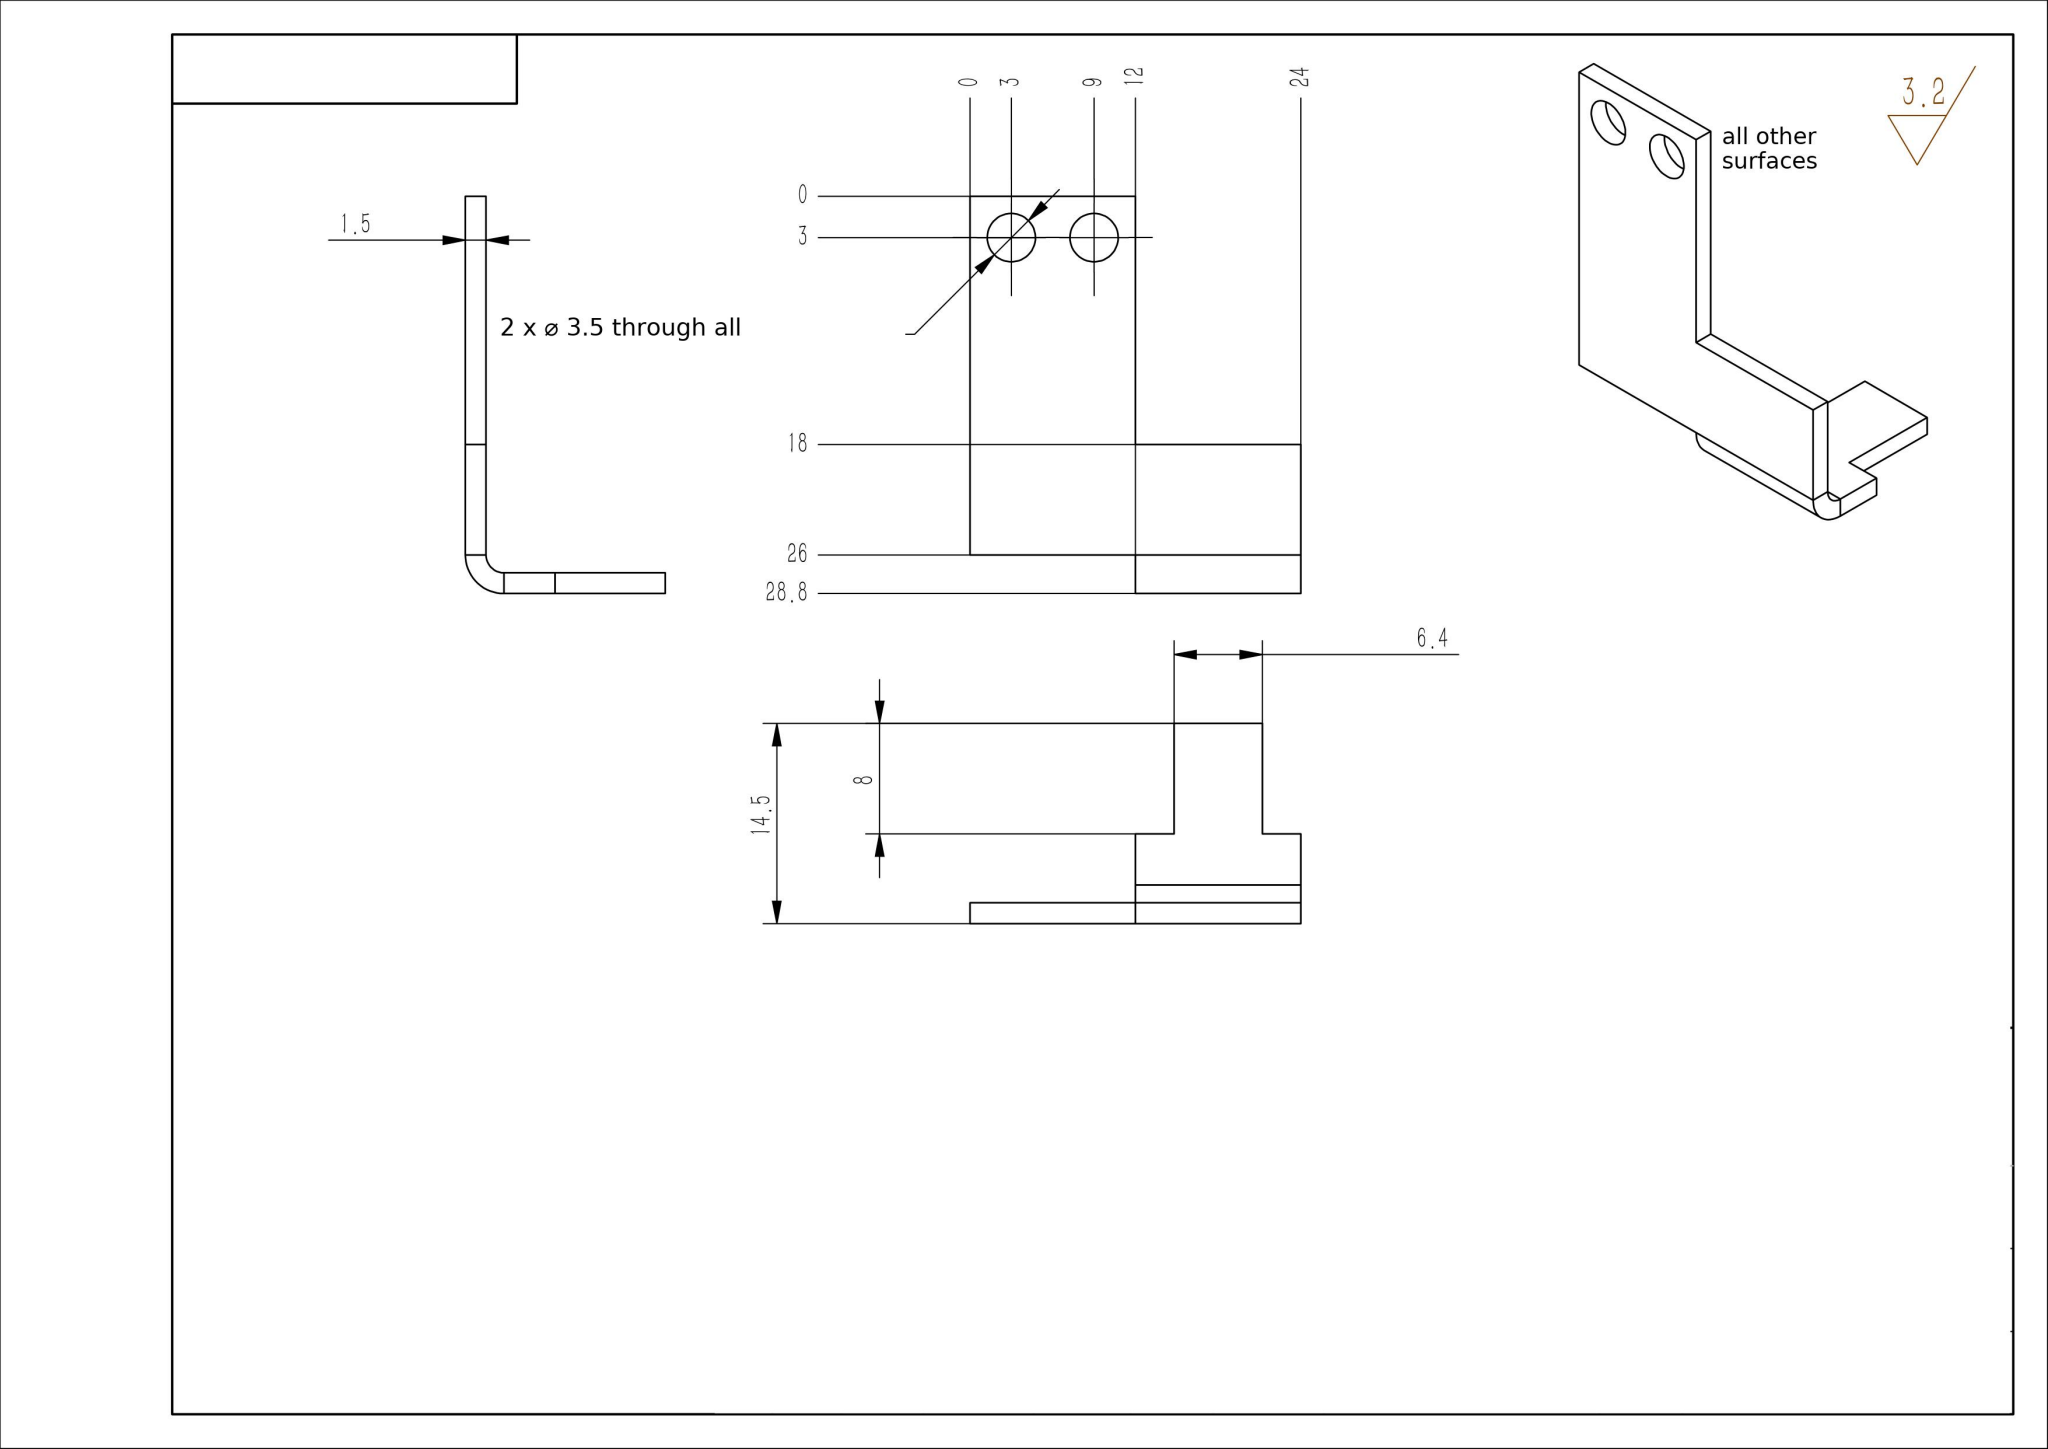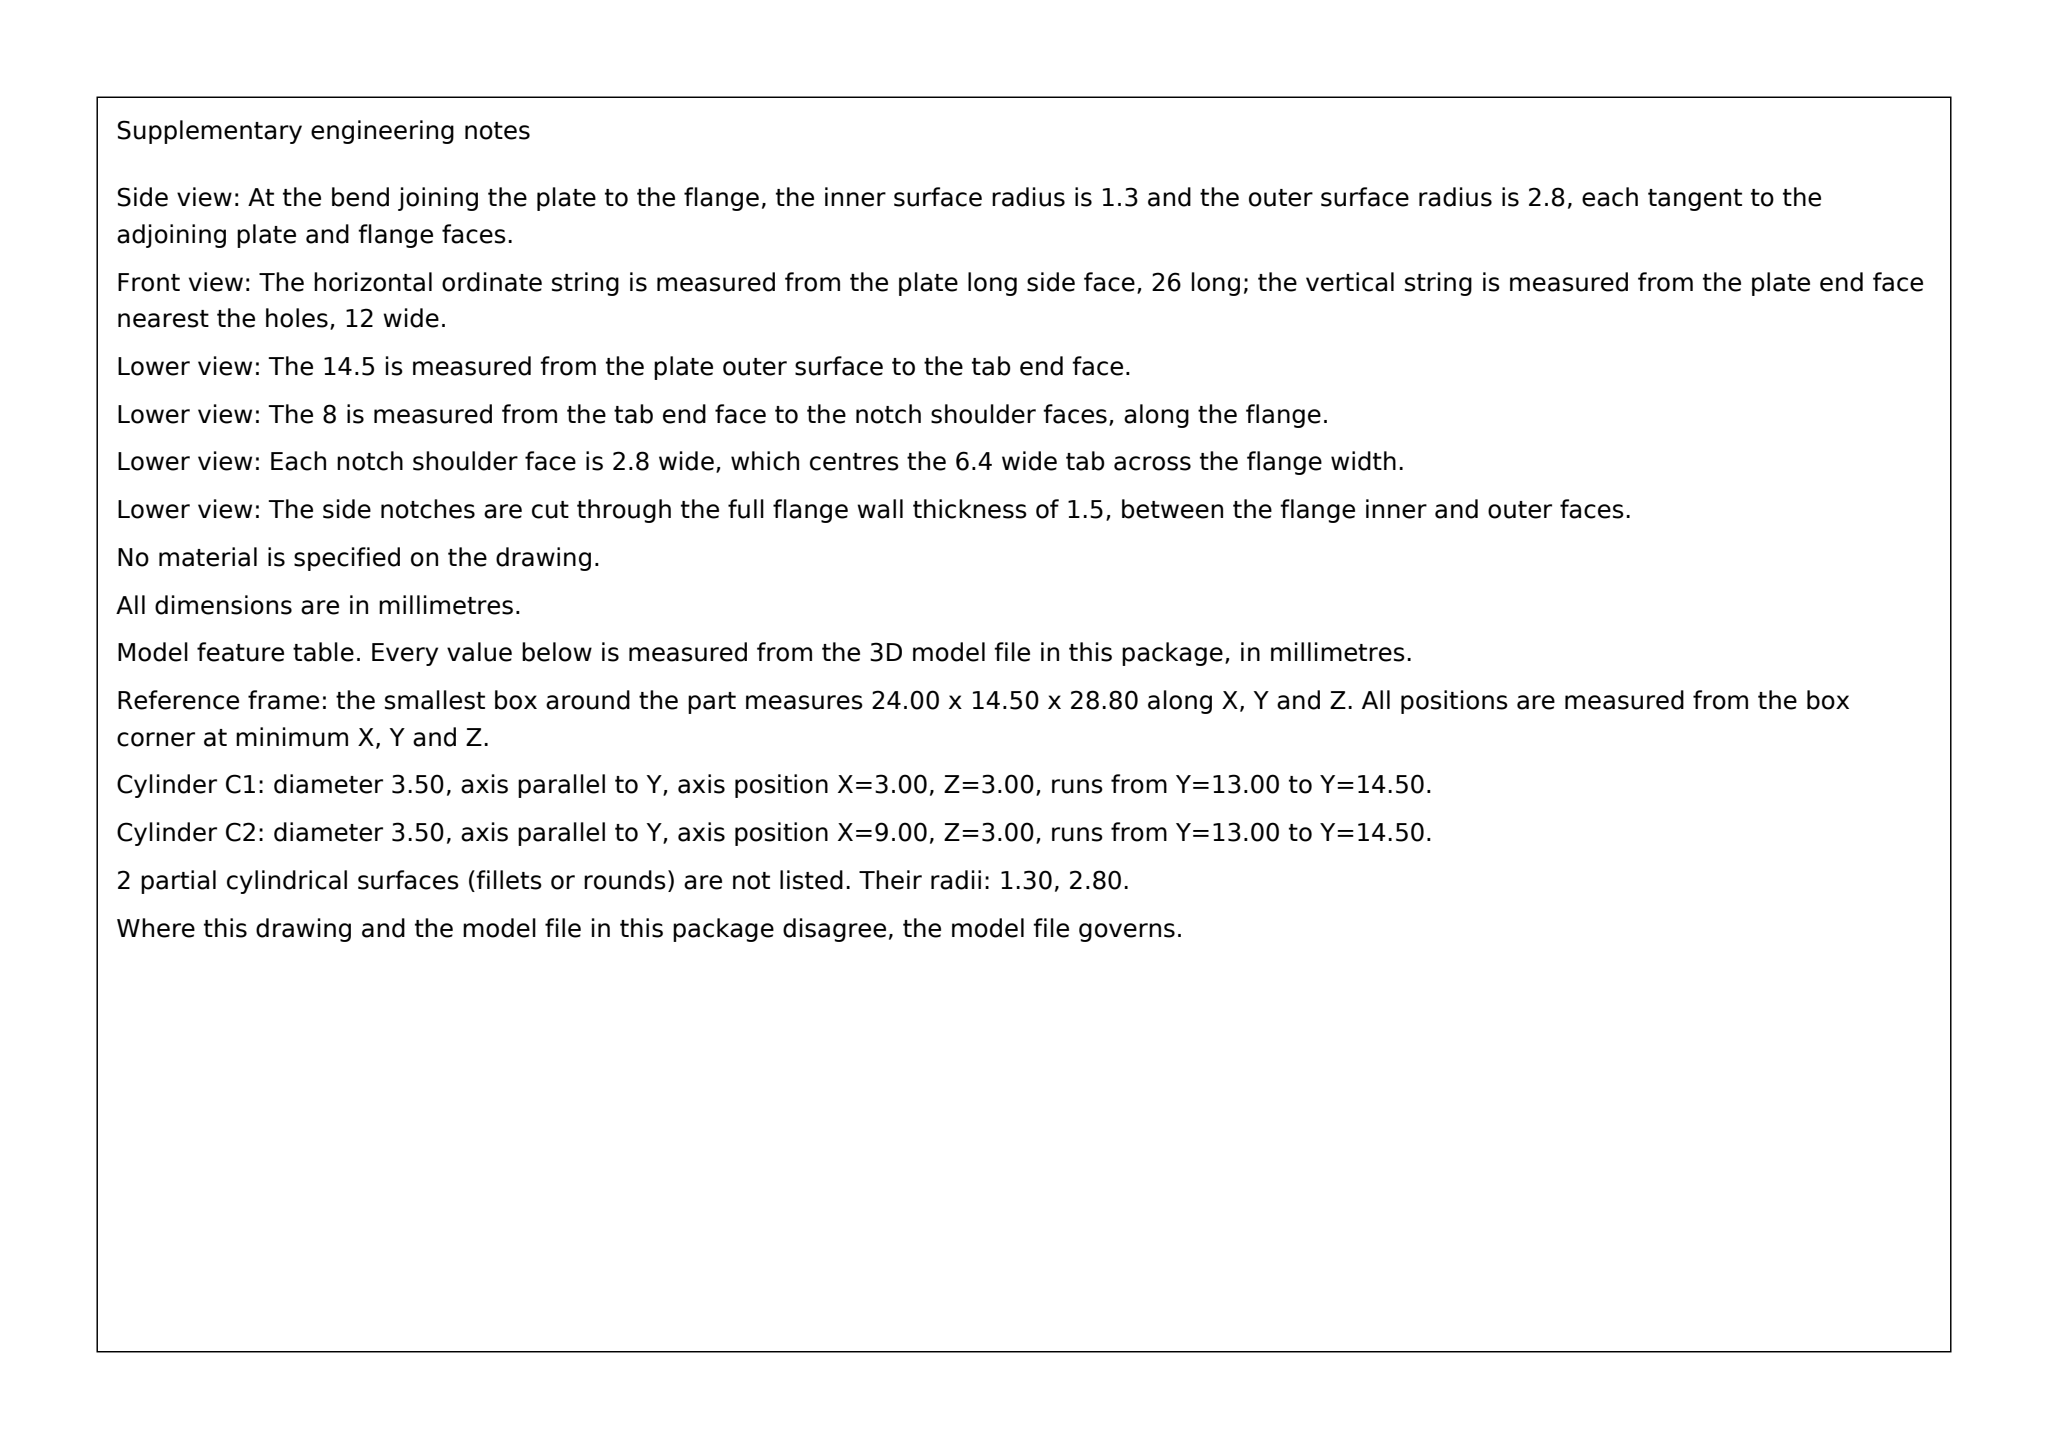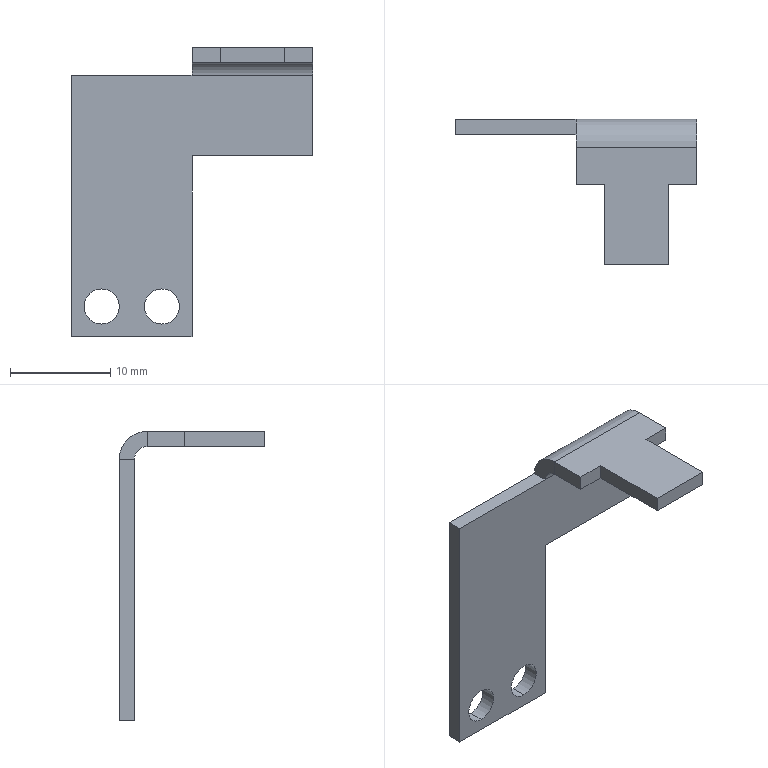Part | SolidWorks | mm | 1 solid | 25 faces | box 24 x 14.5 x 28.8 mm | volume 784 mm3 | plane 19 | cylinder 6 | commonest cylinder face diameters 3.5 x4 5.6 x1 2.6 x1
Drawing notes:
Ø2.6 THRU along X through round end of foot; axis Y11.7, Z26.0 from bbox min corner (hole length 12.0, from X0 to X12) | from the solid: cylinders: [2.6,"x",[null,11.7,26.0],12.0] (its tangent gives the z=27.3 plane)
Ø5.6 round end of foot; axis Y11.7, Z26.0 from bbox min corner, 12.0 long in X | from the solid: cylinders: [5.6,"x",[null,11.7,26.0],12.0]
Axis of Ø5.6/Ø2.6 foot feature located 11.7 from Y0 face (and 26.0 from Z0 datum) | from the solid: cylinders pos_other_axes [null,11.7,26.0]
6.4 wide notch located 14.8 from X0 datum to first wall, 21.2 from X0 datum to second wall (leaves 2.8 to X24 edge) | from the solid: axis_planes x=14.8 and x=21.2, with x=0 and x=24.0 bbox faces
Step face of lower arm/foot at Y8.0 from Y0 datum; plate face at Y13.0, overall part width Y14.5 (1.5 plate thickness) | from the solid: axis_planes y=0.0, y=8.0, y=13.0, y=14.5
ALL DIMENSIONS IN MILLIMETRES | from the solid: STEP model units: mm
FOOT END NOTCH FLOOR AT Z27.3 FROM Z0 DATUM (1.5 DEEP FROM Z28.8 END FACE), 6.4 WIDE FROM X14.8 TO X21.2 | from the solid: axis_planes z offsets 27.3 and 28.8; x offsets 14.8 and 21.2
NOTCH SECOND WALL AT X21.2 FROM X0 DATUM, LEAVING 2.8 OF MATERIAL TO THE X24.0 END FACE | from the solid: axis_planes x offsets 21.2 and 24.0 (bbox_xyz X=24.0)
END-FACE NOTCH: REMAINING WALL 2.8 THICK, FROM X21.2 TO X24.0 END FACE | from the solid: axis_planes x=21.2 and x=24.0 (24.0-21.2=2.8); bbox_xyz x=24.0
STEP:
#1=CARTESIAN_POINT('',(1.,0.,-3.917));
#2=VERTEX_POINT('',#1);
#3=CARTESIAN_POINT('',(1.,0.,-7.417));
#4=VERTEX_POINT('',#3);
#5=CARTESIAN_POINT('',(1.,0.,-5.667));
#6=DIRECTION('',(0.,-1.,0.));
#7=DIRECTION('',(0.,0.,-1.));
#8=AXIS2_PLACEMENT_3D('',#5,#6,#7);
#9=CIRCLE('',#8,1.75);
#10=EDGE_CURVE('',#2,#4,#9,.T.);
#11=ORIENTED_EDGE('',*,*,#10,.F.);
#12=CARTESIAN_POINT('',(1.,-1.5,-3.917));
#13=VERTEX_POINT('',#12);
#14=CARTESIAN_POINT('',(1.,-1.5,-3.917));
#15=DIRECTION('',(0.,-1.,0.));
#16=VECTOR('',#15,1000.);
#17=LINE('',#14,#16);
#18=EDGE_CURVE('',#2,#13,#17,.T.);
#19=ORIENTED_EDGE('',*,*,#18,.T.);
#20=CARTESIAN_POINT('',(1.,-1.5,-7.417));
#21=VERTEX_POINT('',#20);
#22=CARTESIAN_POINT('',(1.,-1.5,-5.667));
#23=DIRECTION('',(0.,-1.,0.));
#24=DIRECTION('',(0.,0.,-1.));
#25=AXIS2_PLACEMENT_3D('',#22,#23,#24);
#26=CIRCLE('',#25,1.75);
#27=EDGE_CURVE('',#13,#21,#26,.T.);
#28=ORIENTED_EDGE('',*,*,#27,.T.);
#29=CARTESIAN_POINT('',(1.,-1.5,-7.417));
#30=DIRECTION('',(0.,-1.,0.));
#31=VECTOR('',#30,1000.);
#32=LINE('',#29,#31);
#33=EDGE_CURVE('',#4,#21,#32,.T.);
#34=ORIENTED_EDGE('',*,*,#33,.F.);
#35=EDGE_LOOP('',(#11,#19,#28,#34));
#36=FACE_OUTER_BOUND('',#35,.T.);
#37=CARTESIAN_POINT('',(1.,-1.5,-5.667));
#38=DIRECTION('',(0.,-1.,0.));
#39=DIRECTION('',(0.,0.,-1.));
#40=AXIS2_PLACEMENT_3D('',#37,#38,#39);
#41=CYLINDRICAL_SURFACE('',#40,1.75);
#42=ADVANCED_FACE('',(#36),#41,.F.);
#43=CARTESIAN_POINT('',(-5.,0.,-3.917));
#44=VERTEX_POINT('',#43);
#45=CARTESIAN_POINT('',(-5.,0.,-7.417));
#46=VERTEX_POINT('',#45);
#47=CARTESIAN_POINT('',(-5.,0.,-5.667));
#48=DIRECTION('',(0.,-1.,0.));
#49=DIRECTION('',(0.,0.,-1.));
#50=AXIS2_PLACEMENT_3D('',#47,#48,#49);
#51=CIRCLE('',#50,1.75);
#52=EDGE_CURVE('',#44,#46,#51,.T.);
#53=ORIENTED_EDGE('',*,*,#52,.F.);
#54=CARTESIAN_POINT('',(-5.,-1.5,-3.917));
#55=VERTEX_POINT('',#54);
#56=CARTESIAN_POINT('',(-5.,-1.5,-3.917));
#57=DIRECTION('',(0.,-1.,0.));
#58=VECTOR('',#57,1000.);
#59=LINE('',#56,#58);
#60=EDGE_CURVE('',#44,#55,#59,.T.);
#61=ORIENTED_EDGE('',*,*,#60,.T.);
#62=CARTESIAN_POINT('',(-5.,-1.5,-7.417));
#63=VERTEX_POINT('',#62);
#64=CARTESIAN_POINT('',(-5.,-1.5,-5.667));
#65=DIRECTION('',(0.,-1.,0.));
#66=DIRECTION('',(0.,0.,-1.));
#67=AXIS2_PLACEMENT_3D('',#64,#65,#66);
#68=CIRCLE('',#67,1.75);
#69=EDGE_CURVE('',#55,#63,#68,.T.);
#70=ORIENTED_EDGE('',*,*,#69,.T.);
#71=CARTESIAN_POINT('',(-5.,-1.5,-7.417));
#72=DIRECTION('',(0.,-1.,0.));
#73=VECTOR('',#72,1000.);
#74=LINE('',#71,#73);
#75=EDGE_CURVE('',#46,#63,#74,.T.);
#76=ORIENTED_EDGE('',*,*,#75,.F.);
#77=EDGE_LOOP('',(#53,#61,#70,#76));
#78=FACE_OUTER_BOUND('',#77,.T.);
#79=CARTESIAN_POINT('',(-5.,-1.5,-5.667));
#80=DIRECTION('',(0.,-1.,0.));
#81=DIRECTION('',(0.,0.,-1.));
#82=AXIS2_PLACEMENT_3D('',#79,#80,#81);
#83=CYLINDRICAL_SURFACE('',#82,1.75);
#84=ADVANCED_FACE('',(#78),#83,.F.);
#85=CARTESIAN_POINT('',(-8.,-1.5,17.333));
#86=VERTEX_POINT('',#85);
#87=CARTESIAN_POINT('',(4.,-1.5,17.333));
#88=VERTEX_POINT('',#87);
#89=CARTESIAN_POINT('',(-8.,-1.5,17.333));
#90=DIRECTION('',(1.,0.,0.));
#91=VECTOR('',#90,1000.);
#92=LINE('',#89,#91);
#93=EDGE_CURVE('',#86,#88,#92,.T.);
#94=ORIENTED_EDGE('',*,*,#93,.T.);
#95=CARTESIAN_POINT('',(4.,0.,17.333));
#96=VERTEX_POINT('',#95);
#97=CARTESIAN_POINT('',(4.,-1.5,17.333));
#98=DIRECTION('',(0.,1.,0.));
#99=VECTOR('',#98,1000.);
#100=LINE('',#97,#99);
#101=EDGE_CURVE('',#88,#96,#100,.T.);
#102=ORIENTED_EDGE('',*,*,#101,.T.);
#103=CARTESIAN_POINT('',(-8.,0.,17.333));
#104=VERTEX_POINT('',#103);
#105=CARTESIAN_POINT('',(-8.,0.,17.333));
#106=DIRECTION('',(1.,0.,0.));
#107=VECTOR('',#106,1000.);
#108=LINE('',#105,#107);
#109=EDGE_CURVE('',#104,#96,#108,.T.);
#110=ORIENTED_EDGE('',*,*,#109,.F.);
#111=CARTESIAN_POINT('',(-8.,-1.5,17.333));
#112=DIRECTION('',(0.,1.,0.));
#113=VECTOR('',#112,1000.);
#114=LINE('',#111,#113);
#115=EDGE_CURVE('',#86,#104,#114,.T.);
#116=ORIENTED_EDGE('',*,*,#115,.F.);
#117=EDGE_LOOP('',(#94,#102,#110,#116));
#118=FACE_OUTER_BOUND('',#117,.T.);
#119=CARTESIAN_POINT('',(-8.,-1.5,17.333));
#120=DIRECTION('',(0.,0.,1.));
#121=DIRECTION('',(1.,0.,0.));
#122=AXIS2_PLACEMENT_3D('',#119,#120,#121);
#123=PLANE('',#122);
#124=ADVANCED_FACE('',(#118),#123,.T.);
#125=CARTESIAN_POINT('',(4.,0.,-8.667));
#126=VERTEX_POINT('',#125);
#127=CARTESIAN_POINT('',(-8.,0.,-8.667));
#128=VERTEX_POINT('',#127);
#129=CARTESIAN_POINT('',(-8.,0.,-8.667));
#130=DIRECTION('',(-1.,0.,0.));
#131=VECTOR('',#130,1000.);
#132=LINE('',#129,#131);
#133=EDGE_CURVE('',#126,#128,#132,.T.);
#134=ORIENTED_EDGE('',*,*,#133,.F.);
#135=CARTESIAN_POINT('',(4.,-1.5,-8.667));
#136=VERTEX_POINT('',#135);
#137=CARTESIAN_POINT('',(4.,-1.5,-8.667));
#138=DIRECTION('',(0.,1.,0.));
#139=VECTOR('',#138,1000.);
#140=LINE('',#137,#139);
#141=EDGE_CURVE('',#136,#126,#140,.T.);
#142=ORIENTED_EDGE('',*,*,#141,.F.);
#143=CARTESIAN_POINT('',(-8.,-1.5,-8.667));
#144=VERTEX_POINT('',#143);
#145=CARTESIAN_POINT('',(-8.,-1.5,-8.667));
#146=DIRECTION('',(-1.,0.,0.));
#147=VECTOR('',#146,1000.);
#148=LINE('',#145,#147);
#149=EDGE_CURVE('',#136,#144,#148,.T.);
#150=ORIENTED_EDGE('',*,*,#149,.T.);
#151=CARTESIAN_POINT('',(-8.,-1.5,-8.667));
#152=DIRECTION('',(0.,1.,0.));
#153=VECTOR('',#152,1000.);
#154=LINE('',#151,#153);
#155=EDGE_CURVE('',#144,#128,#154,.T.);
#156=ORIENTED_EDGE('',*,*,#155,.T.);
#157=EDGE_LOOP('',(#134,#142,#150,#156));
#158=FACE_OUTER_BOUND('',#157,.T.);
#159=CARTESIAN_POINT('',(-8.,-1.5,-8.667));
#160=DIRECTION('',(0.,0.,-1.));
#161=DIRECTION('',(-1.,0.,0.));
#162=AXIS2_PLACEMENT_3D('',#159,#160,#161);
#163=PLANE('',#162);
#164=ADVANCED_FACE('',(#158),#163,.T.);
#165=CARTESIAN_POINT('',(4.,0.,9.333));
#166=VERTEX_POINT('',#165);
#167=CARTESIAN_POINT('',(4.,0.,-8.667));
#168=DIRECTION('',(-0.,0.,-1.));
#169=VECTOR('',#168,1000.);
#170=LINE('',#167,#169);
#171=EDGE_CURVE('',#166,#126,#170,.T.);
#172=ORIENTED_EDGE('',*,*,#171,.F.);
#173=CARTESIAN_POINT('',(4.,-1.5,9.333));
#174=VERTEX_POINT('',#173);
#175=CARTESIAN_POINT('',(4.,-1.5,9.333));
#176=DIRECTION('',(0.,1.,0.));
#177=VECTOR('',#176,1000.);
#178=LINE('',#175,#177);
#179=EDGE_CURVE('',#174,#166,#178,.T.);
#180=ORIENTED_EDGE('',*,*,#179,.F.);
#181=CARTESIAN_POINT('',(4.,-1.5,-8.667));
#182=DIRECTION('',(-0.,0.,-1.));
#183=VECTOR('',#182,1000.);
#184=LINE('',#181,#183);
#185=EDGE_CURVE('',#174,#136,#184,.T.);
#186=ORIENTED_EDGE('',*,*,#185,.T.);
#187=ORIENTED_EDGE('',*,*,#141,.T.);
#188=EDGE_LOOP('',(#172,#180,#186,#187));
#189=FACE_OUTER_BOUND('',#188,.T.);
#190=CARTESIAN_POINT('',(4.,-1.5,-8.667));
#191=DIRECTION('',(1.,0.,-0.));
#192=DIRECTION('',(-0.,0.,-1.));
#193=AXIS2_PLACEMENT_3D('',#190,#191,#192);
#194=PLANE('',#193);
#195=ADVANCED_FACE('',(#189),#194,.T.);
#196=CARTESIAN_POINT('',(16.,0.,9.333));
#197=VERTEX_POINT('',#196);
#198=CARTESIAN_POINT('',(4.,0.,9.333));
#199=DIRECTION('',(-1.,0.,0.));
#200=VECTOR('',#199,1000.);
#201=LINE('',#198,#200);
#202=EDGE_CURVE('',#197,#166,#201,.T.);
#203=ORIENTED_EDGE('',*,*,#202,.F.);
#204=CARTESIAN_POINT('',(16.,-1.5,9.333));
#205=VERTEX_POINT('',#204);
#206=CARTESIAN_POINT('',(16.,-1.5,9.333));
#207=DIRECTION('',(0.,1.,0.));
#208=VECTOR('',#207,1000.);
#209=LINE('',#206,#208);
#210=EDGE_CURVE('',#205,#197,#209,.T.);
#211=ORIENTED_EDGE('',*,*,#210,.F.);
#212=CARTESIAN_POINT('',(4.,-1.5,9.333));
#213=DIRECTION('',(-1.,0.,0.));
#214=VECTOR('',#213,1000.);
#215=LINE('',#212,#214);
#216=EDGE_CURVE('',#205,#174,#215,.T.);
#217=ORIENTED_EDGE('',*,*,#216,.T.);
#218=ORIENTED_EDGE('',*,*,#179,.T.);
#219=EDGE_LOOP('',(#203,#211,#217,#218));
#220=FACE_OUTER_BOUND('',#219,.T.);
#221=CARTESIAN_POINT('',(4.,-1.5,9.333));
#222=DIRECTION('',(0.,0.,-1.));
#223=DIRECTION('',(-1.,0.,0.));
#224=AXIS2_PLACEMENT_3D('',#221,#222,#223);
#225=PLANE('',#224);
#226=ADVANCED_FACE('',(#220),#225,.T.);
#227=CARTESIAN_POINT('',(16.,0.,17.333));
#228=VERTEX_POINT('',#227);
#229=CARTESIAN_POINT('',(16.,0.,9.333));
#230=DIRECTION('',(0.,0.,-1.));
#231=VECTOR('',#230,1000.);
#232=LINE('',#229,#231);
#233=EDGE_CURVE('',#228,#197,#232,.T.);
#234=ORIENTED_EDGE('',*,*,#233,.F.);
#235=CARTESIAN_POINT('',(16.,-1.5,17.333));
#236=VERTEX_POINT('',#235);
#237=CARTESIAN_POINT('',(16.,-1.5,17.333));
#238=DIRECTION('',(0.,1.,0.));
#239=VECTOR('',#238,1000.);
#240=LINE('',#237,#239);
#241=EDGE_CURVE('',#236,#228,#240,.T.);
#242=ORIENTED_EDGE('',*,*,#241,.F.);
#243=CARTESIAN_POINT('',(16.,-1.5,9.333));
#244=DIRECTION('',(0.,0.,-1.));
#245=VECTOR('',#244,1000.);
#246=LINE('',#243,#245);
#247=EDGE_CURVE('',#236,#205,#246,.T.);
#248=ORIENTED_EDGE('',*,*,#247,.T.);
#249=ORIENTED_EDGE('',*,*,#210,.T.);
#250=EDGE_LOOP('',(#234,#242,#248,#249));
#251=FACE_OUTER_BOUND('',#250,.T.);
#252=CARTESIAN_POINT('',(16.,-1.5,9.333));
#253=DIRECTION('',(1.,0.,0.));
#254=DIRECTION('',(0.,0.,-1.));
#255=AXIS2_PLACEMENT_3D('',#252,#253,#254);
#256=PLANE('',#255);
#257=ADVANCED_FACE('',(#251),#256,.T.);
#258=CARTESIAN_POINT('',(-8.,0.,17.333));
#259=DIRECTION('',(0.,0.,1.));
#260=VECTOR('',#259,1000.);
#261=LINE('',#258,#260);
#262=EDGE_CURVE('',#128,#104,#261,.T.);
#263=ORIENTED_EDGE('',*,*,#262,.F.);
#264=ORIENTED_EDGE('',*,*,#155,.F.);
#265=CARTESIAN_POINT('',(-8.,-1.5,17.333));
#266=DIRECTION('',(0.,0.,1.));
#267=VECTOR('',#266,1000.);
#268=LINE('',#265,#267);
#269=EDGE_CURVE('',#144,#86,#268,.T.);
#270=ORIENTED_EDGE('',*,*,#269,.T.);
#271=ORIENTED_EDGE('',*,*,#115,.T.);
#272=EDGE_LOOP('',(#263,#264,#270,#271));
#273=FACE_OUTER_BOUND('',#272,.T.);
#274=CARTESIAN_POINT('',(-8.,-1.5,17.333));
#275=DIRECTION('',(-1.,0.,0.));
#276=DIRECTION('',(0.,0.,1.));
#277=AXIS2_PLACEMENT_3D('',#274,#275,#276);
#278=PLANE('',#277);
#279=ADVANCED_FACE('',(#273),#278,.T.);
#280=CARTESIAN_POINT('',(1.,-1.5,-5.667));
#281=DIRECTION('',(0.,-1.,0.));
#282=DIRECTION('',(0.,0.,-1.));
#283=AXIS2_PLACEMENT_3D('',#280,#281,#282);
#284=CIRCLE('',#283,1.75);
#285=EDGE_CURVE('',#21,#13,#284,.T.);
#286=ORIENTED_EDGE('',*,*,#285,.F.);
#287=ORIENTED_EDGE('',*,*,#27,.F.);
#288=EDGE_LOOP('',(#286,#287));
#289=FACE_BOUND('',#288,.T.);
#290=CARTESIAN_POINT('',(-5.,-1.5,-5.667));
#291=DIRECTION('',(0.,-1.,0.));
#292=DIRECTION('',(0.,0.,-1.));
#293=AXIS2_PLACEMENT_3D('',#290,#291,#292);
#294=CIRCLE('',#293,1.75);
#295=EDGE_CURVE('',#63,#55,#294,.T.);
#296=ORIENTED_EDGE('',*,*,#295,.F.);
#297=ORIENTED_EDGE('',*,*,#69,.F.);
#298=EDGE_LOOP('',(#296,#297));
#299=FACE_BOUND('',#298,.T.);
#300=ORIENTED_EDGE('',*,*,#149,.F.);
#301=ORIENTED_EDGE('',*,*,#185,.F.);
#302=ORIENTED_EDGE('',*,*,#216,.F.);
#303=ORIENTED_EDGE('',*,*,#247,.F.);
#304=CARTESIAN_POINT('',(4.,-1.5,17.333));
#305=DIRECTION('',(1.,0.,0.));
#306=VECTOR('',#305,1000.);
#307=LINE('',#304,#306);
#308=EDGE_CURVE('',#88,#236,#307,.T.);
#309=ORIENTED_EDGE('',*,*,#308,.F.);
#310=ORIENTED_EDGE('',*,*,#93,.F.);
#311=ORIENTED_EDGE('',*,*,#269,.F.);
#312=EDGE_LOOP('',(#300,#301,#302,#303,#309,#310,#311));
#313=FACE_OUTER_BOUND('',#312,.T.);
#314=CARTESIAN_POINT('',(0.,-1.5,0.));
#315=DIRECTION('',(0.,-1.,0.));
#316=DIRECTION('',(0.,0.,-1.));
#317=AXIS2_PLACEMENT_3D('',#314,#315,#316);
#318=PLANE('',#317);
#319=ADVANCED_FACE('',(#289,#299,#313),#318,.T.);
#320=CARTESIAN_POINT('',(1.,0.,-5.667));
#321=DIRECTION('',(0.,-1.,0.));
#322=DIRECTION('',(0.,0.,-1.));
#323=AXIS2_PLACEMENT_3D('',#320,#321,#322);
#324=CIRCLE('',#323,1.75);
#325=EDGE_CURVE('',#4,#2,#324,.T.);
#326=ORIENTED_EDGE('',*,*,#325,.T.);
#327=ORIENTED_EDGE('',*,*,#10,.T.);
#328=EDGE_LOOP('',(#326,#327));
#329=FACE_BOUND('',#328,.T.);
#330=CARTESIAN_POINT('',(-5.,0.,-5.667));
#331=DIRECTION('',(0.,-1.,0.));
#332=DIRECTION('',(0.,0.,-1.));
#333=AXIS2_PLACEMENT_3D('',#330,#331,#332);
#334=CIRCLE('',#333,1.75);
#335=EDGE_CURVE('',#46,#44,#334,.T.);
#336=ORIENTED_EDGE('',*,*,#335,.T.);
#337=ORIENTED_EDGE('',*,*,#52,.T.);
#338=EDGE_LOOP('',(#336,#337));
#339=FACE_BOUND('',#338,.T.);
#340=ORIENTED_EDGE('',*,*,#133,.T.);
#341=ORIENTED_EDGE('',*,*,#262,.T.);
#342=ORIENTED_EDGE('',*,*,#109,.T.);
#343=CARTESIAN_POINT('',(4.,0.,17.333));
#344=DIRECTION('',(1.,0.,0.));
#345=VECTOR('',#344,1000.);
#346=LINE('',#343,#345);
#347=EDGE_CURVE('',#96,#228,#346,.T.);
#348=ORIENTED_EDGE('',*,*,#347,.T.);
#349=ORIENTED_EDGE('',*,*,#233,.T.);
#350=ORIENTED_EDGE('',*,*,#202,.T.);
#351=ORIENTED_EDGE('',*,*,#171,.T.);
#352=EDGE_LOOP('',(#340,#341,#342,#348,#349,#350,#351));
#353=FACE_OUTER_BOUND('',#352,.T.);
#354=CARTESIAN_POINT('',(0.,0.,0.));
#355=DIRECTION('',(0.,-1.,0.));
#356=DIRECTION('',(0.,0.,-1.));
#357=AXIS2_PLACEMENT_3D('',#354,#355,#356);
#358=PLANE('',#357);
#359=ADVANCED_FACE('',(#329,#339,#353),#358,.F.);
#360=CARTESIAN_POINT('',(16.,-2.8,18.633));
#361=VERTEX_POINT('',#360);
#362=CARTESIAN_POINT('',(16.,-2.8,20.133));
#363=VERTEX_POINT('',#362);
#364=CARTESIAN_POINT('',(16.,-2.8,20.133));
#365=DIRECTION('',(0.,0.,1.));
#366=VECTOR('',#365,1000.);
#367=LINE('',#364,#366);
#368=EDGE_CURVE('',#361,#363,#367,.T.);
#369=ORIENTED_EDGE('',*,*,#368,.F.);
#370=CARTESIAN_POINT('',(16.,-2.8,17.333));
#371=DIRECTION('',(1.,0.,0.));
#372=DIRECTION('',(0.,-0.,1.));
#373=AXIS2_PLACEMENT_3D('',#370,#371,#372);
#374=CIRCLE('',#373,1.3);
#375=EDGE_CURVE('',#236,#361,#374,.T.);
#376=ORIENTED_EDGE('',*,*,#375,.F.);
#377=ORIENTED_EDGE('',*,*,#241,.T.);
#378=CARTESIAN_POINT('',(16.,-2.8,17.333));
#379=DIRECTION('',(1.,0.,0.));
#380=DIRECTION('',(0.,-0.,1.));
#381=AXIS2_PLACEMENT_3D('',#378,#379,#380);
#382=CIRCLE('',#381,2.8);
#383=EDGE_CURVE('',#228,#363,#382,.T.);
#384=ORIENTED_EDGE('',*,*,#383,.T.);
#385=EDGE_LOOP('',(#369,#376,#377,#384));
#386=FACE_OUTER_BOUND('',#385,.T.);
#387=CARTESIAN_POINT('',(16.,-2.8,17.333));
#388=DIRECTION('',(1.,0.,0.));
#389=DIRECTION('',(0.,0.,-1.));
#390=AXIS2_PLACEMENT_3D('',#387,#388,#389);
#391=PLANE('',#390);
#392=ADVANCED_FACE('',(#386),#391,.T.);
#393=CARTESIAN_POINT('',(4.,-2.8,18.633));
#394=VERTEX_POINT('',#393);
#395=CARTESIAN_POINT('',(4.,-2.8,17.333));
#396=DIRECTION('',(-1.,0.,0.));
#397=DIRECTION('',(0.,0.,1.));
#398=AXIS2_PLACEMENT_3D('',#395,#396,#397);
#399=CIRCLE('',#398,1.3);
#400=EDGE_CURVE('',#394,#88,#399,.T.);
#401=ORIENTED_EDGE('',*,*,#400,.F.);
#402=CARTESIAN_POINT('',(4.,-2.8,20.133));
#403=VERTEX_POINT('',#402);
#404=CARTESIAN_POINT('',(4.,-2.8,18.633));
#405=DIRECTION('',(0.,0.,1.));
#406=VECTOR('',#405,1000.);
#407=LINE('',#404,#406);
#408=EDGE_CURVE('',#394,#403,#407,.T.);
#409=ORIENTED_EDGE('',*,*,#408,.T.);
#410=CARTESIAN_POINT('',(4.,-2.8,17.333));
#411=DIRECTION('',(-1.,0.,0.));
#412=DIRECTION('',(0.,0.,1.));
#413=AXIS2_PLACEMENT_3D('',#410,#411,#412);
#414=CIRCLE('',#413,2.8);
#415=EDGE_CURVE('',#403,#96,#414,.T.);
#416=ORIENTED_EDGE('',*,*,#415,.T.);
#417=ORIENTED_EDGE('',*,*,#101,.F.);
#418=EDGE_LOOP('',(#401,#409,#416,#417));
#419=FACE_OUTER_BOUND('',#418,.T.);
#420=CARTESIAN_POINT('',(4.,-2.8,17.333));
#421=DIRECTION('',(1.,0.,0.));
#422=DIRECTION('',(0.,0.,-1.));
#423=AXIS2_PLACEMENT_3D('',#420,#421,#422);
#424=PLANE('',#423);
#425=ADVANCED_FACE('',(#419),#424,.F.);
#426=ORIENTED_EDGE('',*,*,#347,.F.);
#427=ORIENTED_EDGE('',*,*,#415,.F.);
#428=CARTESIAN_POINT('',(0.,-2.8,20.133));
#429=DIRECTION('',(-1.,0.,0.));
#430=VECTOR('',#429,1000.);
#431=LINE('',#428,#430);
#432=EDGE_CURVE('',#363,#403,#431,.T.);
#433=ORIENTED_EDGE('',*,*,#432,.F.);
#434=ORIENTED_EDGE('',*,*,#383,.F.);
#435=EDGE_LOOP('',(#426,#427,#433,#434));
#436=FACE_OUTER_BOUND('',#435,.T.);
#437=CARTESIAN_POINT('',(4.,-2.8,17.333));
#438=DIRECTION('',(-1.,0.,0.));
#439=DIRECTION('',(0.,0.,1.));
#440=AXIS2_PLACEMENT_3D('',#437,#438,#439);
#441=CYLINDRICAL_SURFACE('',#440,2.8);
#442=ADVANCED_FACE('',(#436),#441,.T.);
#443=ORIENTED_EDGE('',*,*,#308,.T.);
#444=ORIENTED_EDGE('',*,*,#375,.T.);
#445=CARTESIAN_POINT('',(16.,-2.8,18.633));
#446=DIRECTION('',(-1.,0.,0.));
#447=VECTOR('',#446,1000.);
#448=LINE('',#445,#447);
#449=EDGE_CURVE('',#361,#394,#448,.T.);
#450=ORIENTED_EDGE('',*,*,#449,.T.);
#451=ORIENTED_EDGE('',*,*,#400,.T.);
#452=EDGE_LOOP('',(#443,#444,#450,#451));
#453=FACE_OUTER_BOUND('',#452,.T.);
#454=CARTESIAN_POINT('',(4.,-2.8,17.333));
#455=DIRECTION('',(-1.,0.,0.));
#456=DIRECTION('',(0.,0.,1.));
#457=AXIS2_PLACEMENT_3D('',#454,#455,#456);
#458=CYLINDRICAL_SURFACE('',#457,1.3);
#459=ADVANCED_FACE('',(#453),#458,.F.);
#460=CARTESIAN_POINT('',(4.,-6.5,20.133));
#461=VERTEX_POINT('',#460);
#462=CARTESIAN_POINT('',(4.,-6.5,18.633));
#463=VERTEX_POINT('',#462);
#464=CARTESIAN_POINT('',(4.,-6.5,20.133));
#465=DIRECTION('',(0.,-0.,-1.));
#466=VECTOR('',#465,1000.);
#467=LINE('',#464,#466);
#468=EDGE_CURVE('',#461,#463,#467,.T.);
#469=ORIENTED_EDGE('',*,*,#468,.F.);
#470=CARTESIAN_POINT('',(4.,-1.5,20.133));
#471=DIRECTION('',(0.,1.,-0.));
#472=VECTOR('',#471,1000.);
#473=LINE('',#470,#472);
#474=EDGE_CURVE('',#461,#403,#473,.T.);
#475=ORIENTED_EDGE('',*,*,#474,.T.);
#476=ORIENTED_EDGE('',*,*,#408,.F.);
#477=CARTESIAN_POINT('',(4.,0.,18.633));
#478=DIRECTION('',(0.,1.,-0.));
#479=VECTOR('',#478,1000.);
#480=LINE('',#477,#479);
#481=EDGE_CURVE('',#463,#394,#480,.T.);
#482=ORIENTED_EDGE('',*,*,#481,.F.);
#483=EDGE_LOOP('',(#469,#475,#476,#482));
#484=FACE_OUTER_BOUND('',#483,.T.);
#485=CARTESIAN_POINT('',(4.,-1.5,20.133));
#486=DIRECTION('',(-1.,0.,0.));
#487=DIRECTION('',(0.,0.,1.));
#488=AXIS2_PLACEMENT_3D('',#485,#486,#487);
#489=PLANE('',#488);
#490=ADVANCED_FACE('',(#484),#489,.T.);
#491=CARTESIAN_POINT('',(16.,-6.5,18.633));
#492=VERTEX_POINT('',#491);
#493=CARTESIAN_POINT('',(16.,-6.5,20.133));
#494=VERTEX_POINT('',#493);
#495=CARTESIAN_POINT('',(16.,-6.5,20.133));
#496=DIRECTION('',(0.,0.,1.));
#497=VECTOR('',#496,1000.);
#498=LINE('',#495,#497);
#499=EDGE_CURVE('',#492,#494,#498,.T.);
#500=ORIENTED_EDGE('',*,*,#499,.F.);
#501=CARTESIAN_POINT('',(16.,0.,18.633));
#502=DIRECTION('',(0.,-1.,0.));
#503=VECTOR('',#502,1000.);
#504=LINE('',#501,#503);
#505=EDGE_CURVE('',#361,#492,#504,.T.);
#506=ORIENTED_EDGE('',*,*,#505,.F.);
#507=ORIENTED_EDGE('',*,*,#368,.T.);
#508=CARTESIAN_POINT('',(16.,-14.5,20.133));
#509=DIRECTION('',(0.,-1.,0.));
#510=VECTOR('',#509,1000.);
#511=LINE('',#508,#510);
#512=EDGE_CURVE('',#363,#494,#511,.T.);
#513=ORIENTED_EDGE('',*,*,#512,.T.);
#514=EDGE_LOOP('',(#500,#506,#507,#513));
#515=FACE_OUTER_BOUND('',#514,.T.);
#516=CARTESIAN_POINT('',(16.,-14.5,20.133));
#517=DIRECTION('',(1.,0.,0.));
#518=DIRECTION('',(0.,0.,-1.));
#519=AXIS2_PLACEMENT_3D('',#516,#517,#518);
#520=PLANE('',#519);
#521=ADVANCED_FACE('',(#515),#520,.T.);
#522=CARTESIAN_POINT('',(6.8,-6.5,20.133));
#523=VERTEX_POINT('',#522);
#524=CARTESIAN_POINT('',(0.,-6.5,20.133));
#525=DIRECTION('',(-1.,0.,0.));
#526=VECTOR('',#525,1000.);
#527=LINE('',#524,#526);
#528=EDGE_CURVE('',#523,#461,#527,.T.);
#529=ORIENTED_EDGE('',*,*,#528,.F.);
#530=CARTESIAN_POINT('',(6.8,-14.5,20.133));
#531=VERTEX_POINT('',#530);
#532=CARTESIAN_POINT('',(6.8,0.,20.133));
#533=DIRECTION('',(-0.,1.,-0.));
#534=VECTOR('',#533,1000.);
#535=LINE('',#532,#534);
#536=EDGE_CURVE('',#531,#523,#535,.T.);
#537=ORIENTED_EDGE('',*,*,#536,.F.);
#538=CARTESIAN_POINT('',(13.2,-14.5,20.133));
#539=VERTEX_POINT('',#538);
#540=CARTESIAN_POINT('',(4.,-14.5,20.133));
#541=DIRECTION('',(-1.,0.,0.));
#542=VECTOR('',#541,1000.);
#543=LINE('',#540,#542);
#544=EDGE_CURVE('',#539,#531,#543,.T.);
#545=ORIENTED_EDGE('',*,*,#544,.F.);
#546=CARTESIAN_POINT('',(13.2,-6.5,20.133));
#547=VERTEX_POINT('',#546);
#548=CARTESIAN_POINT('',(13.2,0.,20.133));
#549=DIRECTION('',(0.,-1.,0.));
#550=VECTOR('',#549,1000.);
#551=LINE('',#548,#550);
#552=EDGE_CURVE('',#547,#539,#551,.T.);
#553=ORIENTED_EDGE('',*,*,#552,.F.);
#554=CARTESIAN_POINT('',(0.,-6.5,20.133));
#555=DIRECTION('',(-1.,0.,0.));
#556=VECTOR('',#555,1000.);
#557=LINE('',#554,#556);
#558=EDGE_CURVE('',#494,#547,#557,.T.);
#559=ORIENTED_EDGE('',*,*,#558,.F.);
#560=ORIENTED_EDGE('',*,*,#512,.F.);
#561=ORIENTED_EDGE('',*,*,#432,.T.);
#562=ORIENTED_EDGE('',*,*,#474,.F.);
#563=EDGE_LOOP('',(#529,#537,#545,#553,#559,#560,#561,#562));
#564=FACE_OUTER_BOUND('',#563,.T.);
#565=CARTESIAN_POINT('',(0.,0.,20.133));
#566=DIRECTION('',(0.,0.,1.));
#567=DIRECTION('',(0.,-1.,0.));
#568=AXIS2_PLACEMENT_3D('',#565,#566,#567);
#569=PLANE('',#568);
#570=ADVANCED_FACE('',(#564),#569,.T.);
#571=CARTESIAN_POINT('',(6.8,-6.5,18.633));
#572=VERTEX_POINT('',#571);
#573=CARTESIAN_POINT('',(6.8,-14.5,18.633));
#574=VERTEX_POINT('',#573);
#575=CARTESIAN_POINT('',(6.8,-6.5,18.633));
#576=DIRECTION('',(0.,-1.,0.));
#577=VECTOR('',#576,1000.);
#578=LINE('',#575,#577);
#579=EDGE_CURVE('',#572,#574,#578,.T.);
#580=ORIENTED_EDGE('',*,*,#579,.F.);
#581=CARTESIAN_POINT('',(1.964,-6.5,18.633));
#582=DIRECTION('',(1.,0.,0.));
#583=VECTOR('',#582,1000.);
#584=LINE('',#581,#583);
#585=EDGE_CURVE('',#463,#572,#584,.T.);
#586=ORIENTED_EDGE('',*,*,#585,.F.);
#587=ORIENTED_EDGE('',*,*,#481,.T.);
#588=ORIENTED_EDGE('',*,*,#449,.F.);
#589=ORIENTED_EDGE('',*,*,#505,.T.);
#590=CARTESIAN_POINT('',(13.2,-6.5,18.633));
#591=VERTEX_POINT('',#590);
#592=CARTESIAN_POINT('',(18.036,-6.5,18.633));
#593=DIRECTION('',(1.,0.,0.));
#594=VECTOR('',#593,1000.);
#595=LINE('',#592,#594);
#596=EDGE_CURVE('',#591,#492,#595,.T.);
#597=ORIENTED_EDGE('',*,*,#596,.F.);
#598=CARTESIAN_POINT('',(13.2,-14.5,18.633));
#599=VERTEX_POINT('',#598);
#600=CARTESIAN_POINT('',(13.2,-6.5,18.633));
#601=DIRECTION('',(0.,1.,-0.));
#602=VECTOR('',#601,1000.);
#603=LINE('',#600,#602);
#604=EDGE_CURVE('',#599,#591,#603,.T.);
#605=ORIENTED_EDGE('',*,*,#604,.F.);
#606=CARTESIAN_POINT('',(0.,-14.5,18.633));
#607=DIRECTION('',(-1.,0.,0.));
#608=VECTOR('',#607,1000.);
#609=LINE('',#606,#608);
#610=EDGE_CURVE('',#599,#574,#609,.T.);
#611=ORIENTED_EDGE('',*,*,#610,.T.);
#612=EDGE_LOOP('',(#580,#586,#587,#588,#589,#597,#605,#611));
#613=FACE_OUTER_BOUND('',#612,.T.);
#614=CARTESIAN_POINT('',(0.,0.,18.633));
#615=DIRECTION('',(0.,0.,1.));
#616=DIRECTION('',(0.,-1.,0.));
#617=AXIS2_PLACEMENT_3D('',#614,#615,#616);
#618=PLANE('',#617);
#619=ADVANCED_FACE('',(#613),#618,.F.);
#620=CARTESIAN_POINT('',(6.8,-14.5,20.133));
#621=DIRECTION('',(-0.,0.,1.));
#622=VECTOR('',#621,1000.);
#623=LINE('',#620,#622);
#624=EDGE_CURVE('',#574,#531,#623,.T.);
#625=ORIENTED_EDGE('',*,*,#624,.F.);
#626=ORIENTED_EDGE('',*,*,#610,.F.);
#627=CARTESIAN_POINT('',(13.2,-14.5,20.133));
#628=DIRECTION('',(0.,-0.,-1.));
#629=VECTOR('',#628,1000.);
#630=LINE('',#627,#629);
#631=EDGE_CURVE('',#539,#599,#630,.T.);
#632=ORIENTED_EDGE('',*,*,#631,.F.);
#633=ORIENTED_EDGE('',*,*,#544,.T.);
#634=EDGE_LOOP('',(#625,#626,#632,#633));
#635=FACE_OUTER_BOUND('',#634,.T.);
#636=CARTESIAN_POINT('',(4.,-14.5,20.133));
#637=DIRECTION('',(0.,-1.,0.));
#638=DIRECTION('',(0.,-0.,-1.));
#639=AXIS2_PLACEMENT_3D('',#636,#637,#638);
#640=PLANE('',#639);
#641=ADVANCED_FACE('',(#635),#640,.T.);
#642=ORIENTED_EDGE('',*,*,#499,.T.);
#643=ORIENTED_EDGE('',*,*,#558,.T.);
#644=CARTESIAN_POINT('',(13.2,-6.5,20.133));
#645=DIRECTION('',(0.,-0.,-1.));
#646=VECTOR('',#645,1000.);
#647=LINE('',#644,#646);
#648=EDGE_CURVE('',#547,#591,#647,.T.);
#649=ORIENTED_EDGE('',*,*,#648,.T.);
#650=ORIENTED_EDGE('',*,*,#596,.T.);
#651=EDGE_LOOP('',(#642,#643,#649,#650));
#652=FACE_OUTER_BOUND('',#651,.T.);
#653=CARTESIAN_POINT('',(18.036,-6.5,20.133));
#654=DIRECTION('',(0.,1.,-0.));
#655=DIRECTION('',(0.,0.,1.));
#656=AXIS2_PLACEMENT_3D('',#653,#654,#655);
#657=PLANE('',#656);
#658=ADVANCED_FACE('',(#652),#657,.F.);
#659=ORIENTED_EDGE('',*,*,#552,.T.);
#660=ORIENTED_EDGE('',*,*,#631,.T.);
#661=ORIENTED_EDGE('',*,*,#604,.T.);
#662=ORIENTED_EDGE('',*,*,#648,.F.);
#663=EDGE_LOOP('',(#659,#660,#661,#662));
#664=FACE_OUTER_BOUND('',#663,.T.);
#665=CARTESIAN_POINT('',(13.2,-6.5,20.133));
#666=DIRECTION('',(-1.,0.,0.));
#667=DIRECTION('',(0.,0.,1.));
#668=AXIS2_PLACEMENT_3D('',#665,#666,#667);
#669=PLANE('',#668);
#670=ADVANCED_FACE('',(#664),#669,.F.);
#671=ORIENTED_EDGE('',*,*,#468,.T.);
#672=ORIENTED_EDGE('',*,*,#585,.T.);
#673=CARTESIAN_POINT('',(6.8,-6.5,20.133));
#674=DIRECTION('',(0.,-0.,-1.));
#675=VECTOR('',#674,1000.);
#676=LINE('',#673,#675);
#677=EDGE_CURVE('',#523,#572,#676,.T.);
#678=ORIENTED_EDGE('',*,*,#677,.F.);
#679=ORIENTED_EDGE('',*,*,#528,.T.);
#680=EDGE_LOOP('',(#671,#672,#678,#679));
#681=FACE_OUTER_BOUND('',#680,.T.);
#682=CARTESIAN_POINT('',(1.964,-6.5,20.133));
#683=DIRECTION('',(0.,1.,-0.));
#684=DIRECTION('',(0.,0.,1.));
#685=AXIS2_PLACEMENT_3D('',#682,#683,#684);
#686=PLANE('',#685);
#687=ADVANCED_FACE('',(#681),#686,.F.);
#688=ORIENTED_EDGE('',*,*,#536,.T.);
#689=ORIENTED_EDGE('',*,*,#677,.T.);
#690=ORIENTED_EDGE('',*,*,#579,.T.);
#691=ORIENTED_EDGE('',*,*,#624,.T.);
#692=EDGE_LOOP('',(#688,#689,#690,#691));
#693=FACE_OUTER_BOUND('',#692,.T.);
#694=CARTESIAN_POINT('',(6.8,-6.5,20.133));
#695=DIRECTION('',(1.,0.,-0.));
#696=DIRECTION('',(-0.,1.,0.));
#697=AXIS2_PLACEMENT_3D('',#694,#695,#696);
#698=PLANE('',#697);
#699=ADVANCED_FACE('',(#693),#698,.F.);
#700=ORIENTED_EDGE('',*,*,#60,.F.);
#701=ORIENTED_EDGE('',*,*,#335,.F.);
#702=ORIENTED_EDGE('',*,*,#75,.T.);
#703=ORIENTED_EDGE('',*,*,#295,.T.);
#704=EDGE_LOOP('',(#700,#701,#702,#703));
#705=FACE_OUTER_BOUND('',#704,.T.);
#706=CARTESIAN_POINT('',(-5.,-1.5,-5.667));
#707=DIRECTION('',(0.,-1.,0.));
#708=DIRECTION('',(0.,0.,-1.));
#709=AXIS2_PLACEMENT_3D('',#706,#707,#708);
#710=CYLINDRICAL_SURFACE('',#709,1.75);
#711=ADVANCED_FACE('',(#705),#710,.F.);
#712=ORIENTED_EDGE('',*,*,#18,.F.);
#713=ORIENTED_EDGE('',*,*,#325,.F.);
#714=ORIENTED_EDGE('',*,*,#33,.T.);
#715=ORIENTED_EDGE('',*,*,#285,.T.);
#716=EDGE_LOOP('',(#712,#713,#714,#715));
#717=FACE_OUTER_BOUND('',#716,.T.);
#718=CARTESIAN_POINT('',(1.,-1.5,-5.667));
#719=DIRECTION('',(0.,-1.,0.));
#720=DIRECTION('',(0.,0.,-1.));
#721=AXIS2_PLACEMENT_3D('',#718,#719,#720);
#722=CYLINDRICAL_SURFACE('',#721,1.75);
#723=ADVANCED_FACE('',(#717),#722,.F.);
#724=CLOSED_SHELL('',(#42,#84,#124,#164,#195,#226,#257,#279,#319,#359,#392,#425,#442,#459,#490,#521,#570,#619,#641,#658,#670,#687,#699,#711,#723));
#725=MANIFOLD_SOLID_BREP('',#724);
#726=CARTESIAN_POINT('',(0.,0.,0.));
#727=DIRECTION('',(0.,0.,1.));
#728=DIRECTION('',(1.,0.,0.));
#729=AXIS2_PLACEMENT_3D('',#726,#727,#728);
#730=(LENGTH_UNIT()NAMED_UNIT(*)SI_UNIT(.MILLI.,.METRE.));
#731=UNCERTAINTY_MEASURE_WITH_UNIT(LENGTH_MEASURE(0.00001),#730,'','');
#732=(NAMED_UNIT(*)PLANE_ANGLE_UNIT()SI_UNIT($,.RADIAN.));
#733=(NAMED_UNIT(*)SI_UNIT($,.STERADIAN.)SOLID_ANGLE_UNIT());
#734=(GEOMETRIC_REPRESENTATION_CONTEXT(3)GLOBAL_UNCERTAINTY_ASSIGNED_CONTEXT((#731))GLOBAL_UNIT_ASSIGNED_CONTEXT((#730,#732,#733))REPRESENTATION_CONTEXT('',''));
#735=ADVANCED_BREP_SHAPE_REPRESENTATION('',(#725,#729),#734);